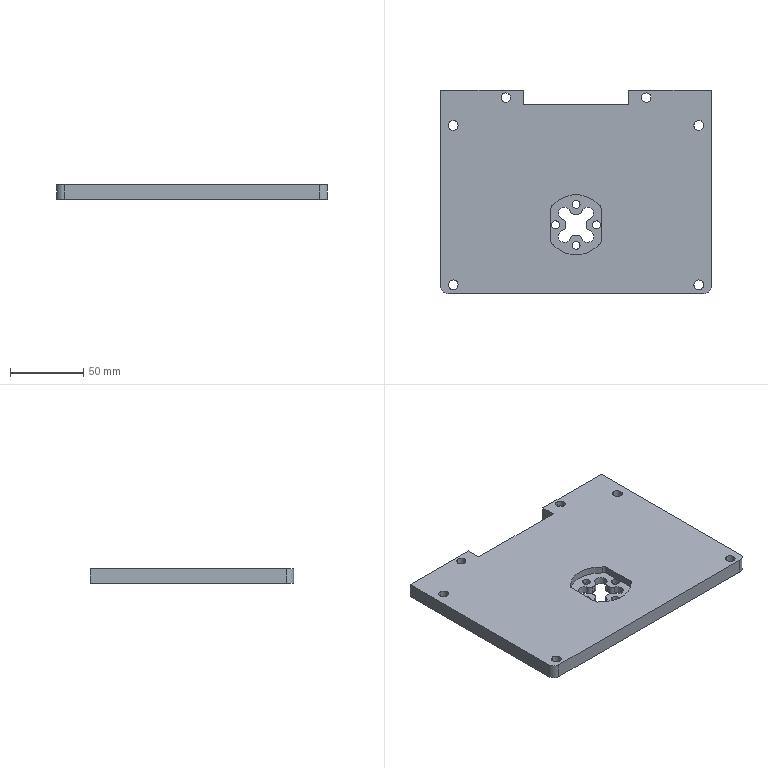CAM job | Mastercam | mm | 18 operations | part box 185 x 139 x 10
1. Contour (Ramp) | 10 - 10 平铣刀
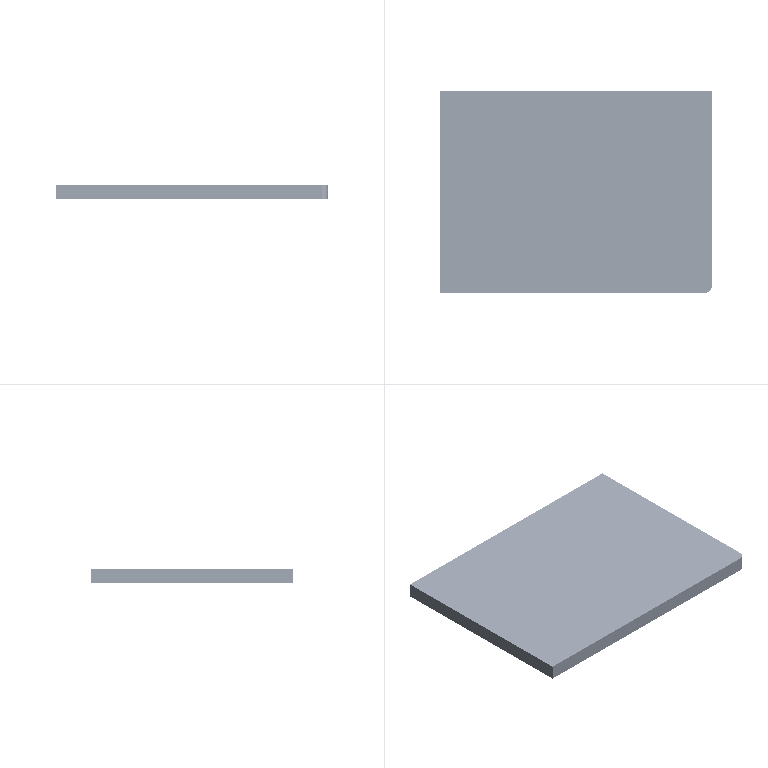2. Contour (2D) | 10 - 10 平铣刀
3. Contour (Ramp) | 10 - 10 平铣刀
4. Contour (Ramp) | 10 - 10 平铣刀
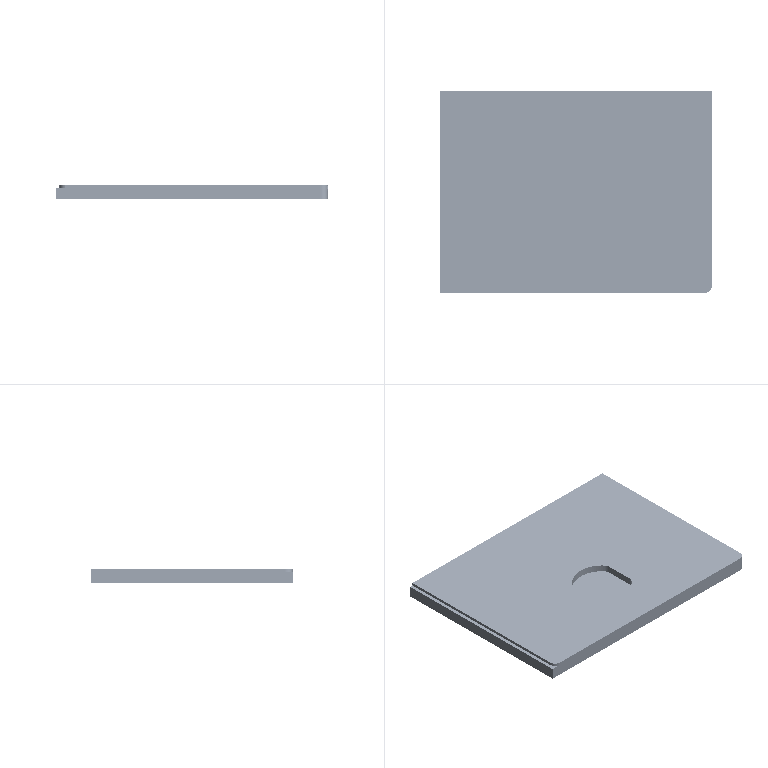5. Contour (Ramp) | 5 - 5 平铣刀
6. Contour (Ramp) | 5 - 5 平铣刀
7. Contour (Remachining) | 5 - 5 平铣刀
8. 2D High Speed (2D Area Mill) | 5 - 5 平铣刀
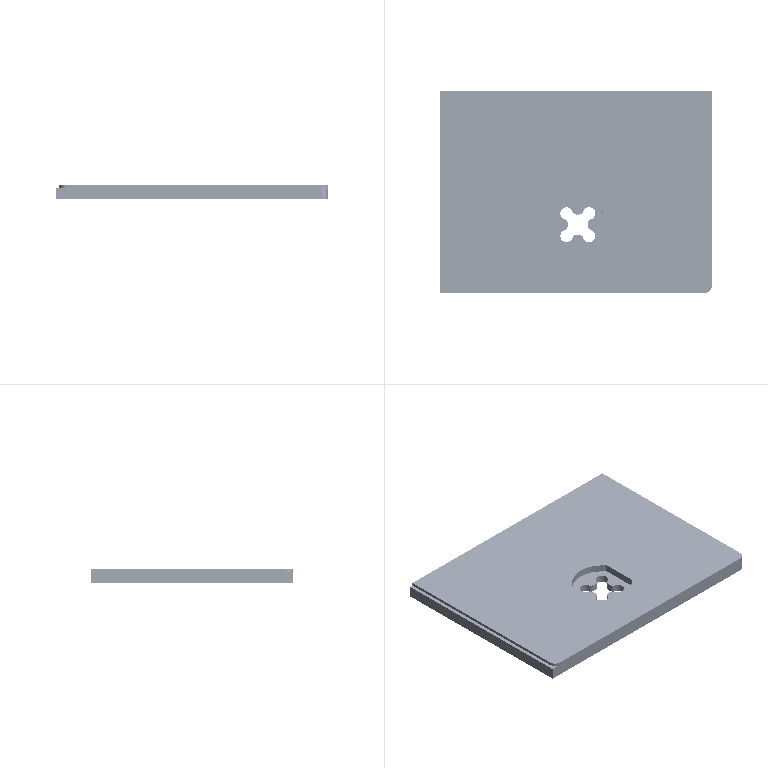9. Contour (2D) | 5 - 5 平铣刀
10. Drill/Counterbore | 7 - 4 倒角刀
11. Contour (2D chamfer) | 7 - 4 倒角刀
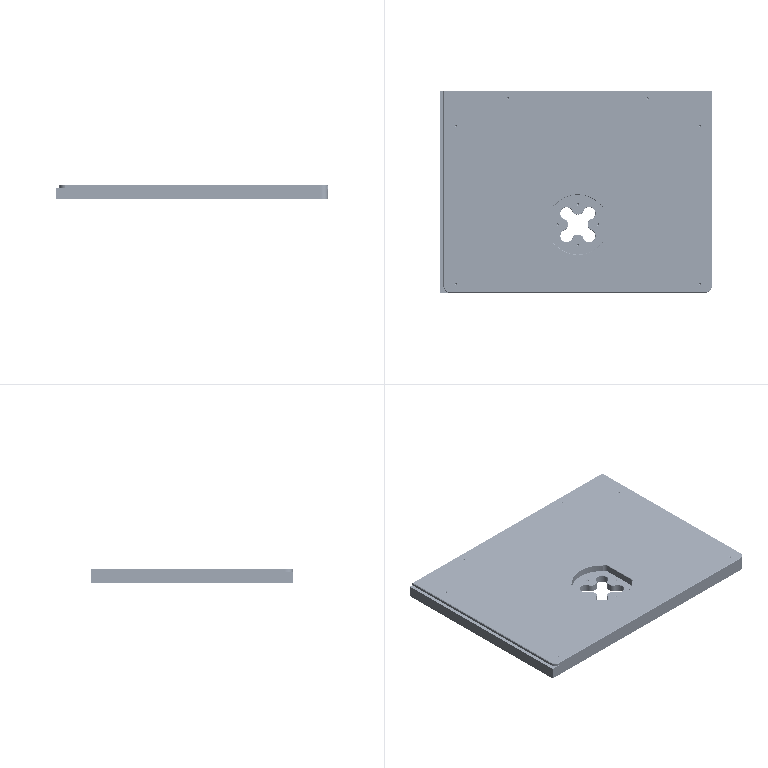12. Contour (Ramp) | 10 - 10 平铣刀
13. Contour (2D) | 10 - 10 平铣刀
14. Contour (Ramp) | 6 - 6 平铣刀
15. Contour (2D) | 6 - 6 平铣刀
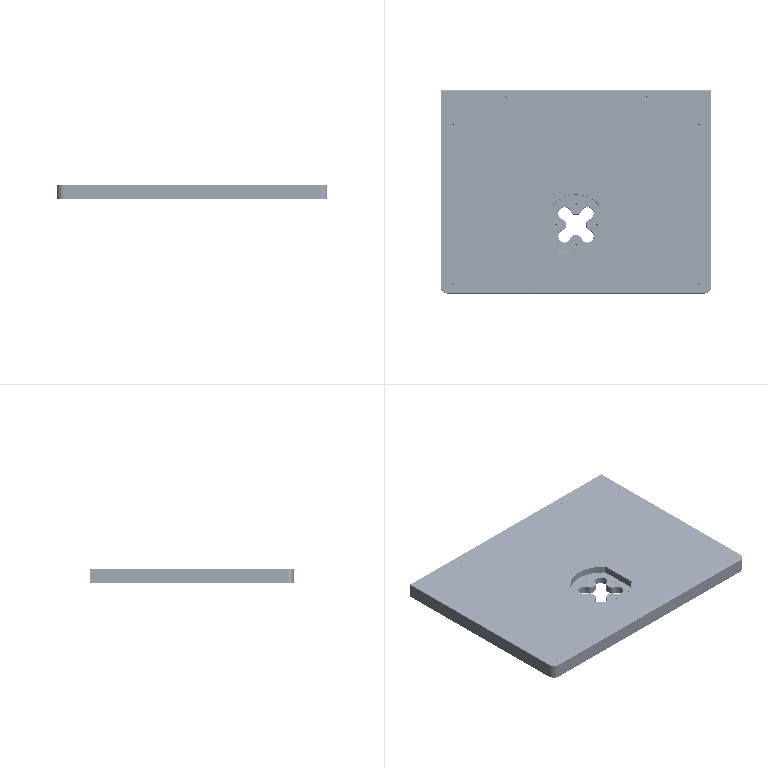16. Contour (2D chamfer) | 7 - 4 倒角刀
17. Contour (Ramp) | 10 - 10 平铣刀
18. Contour (2D) | 10 - 10 平铣刀